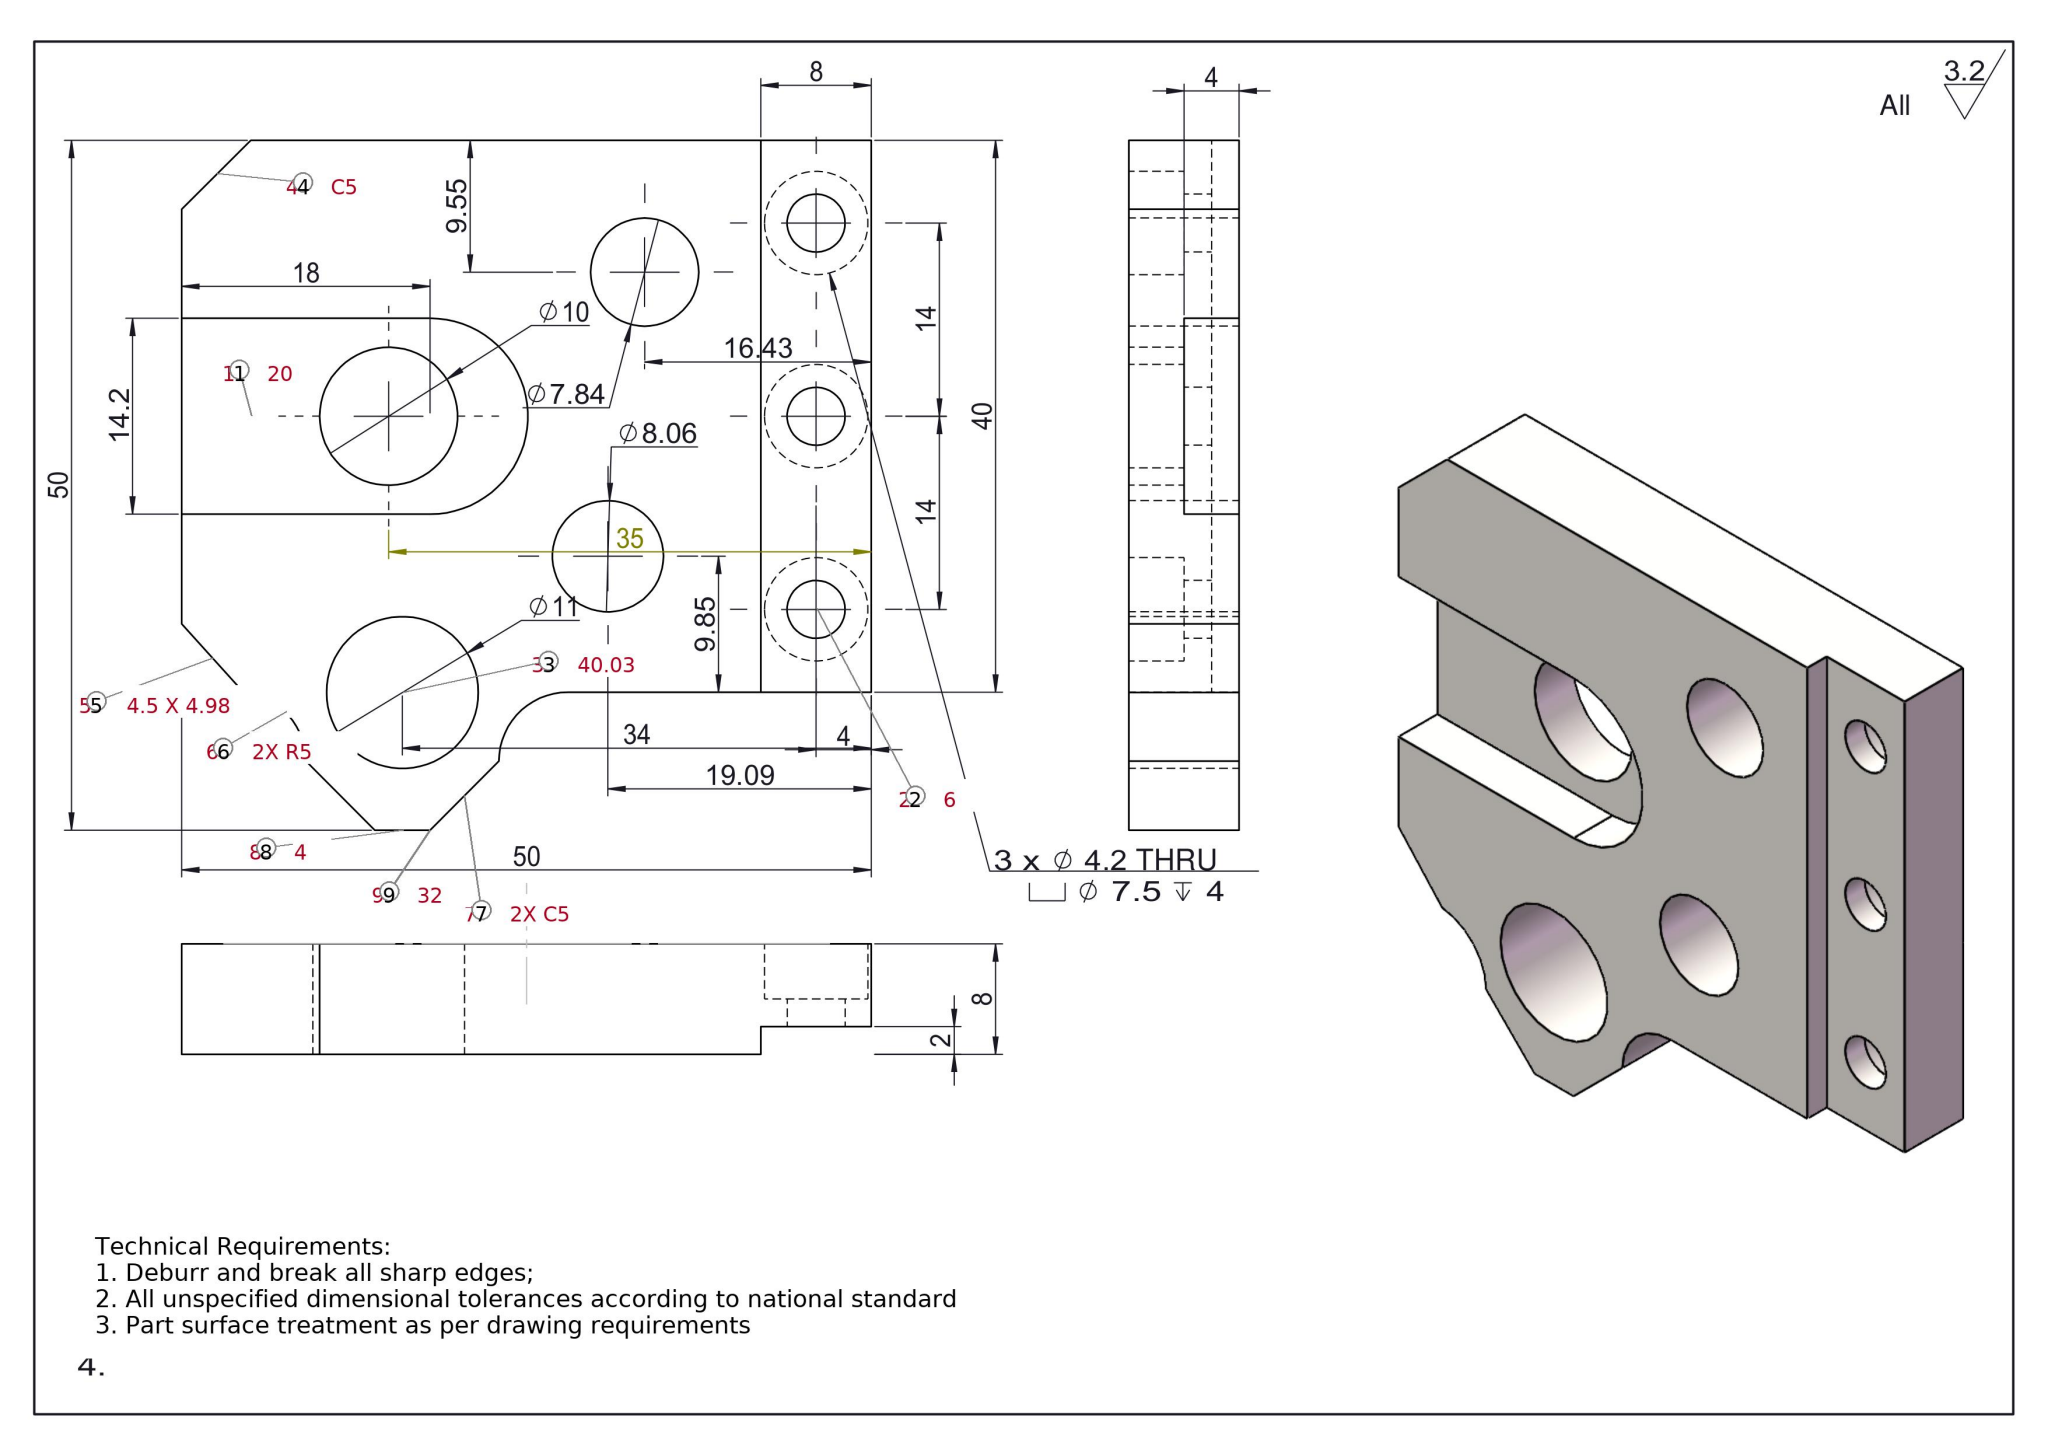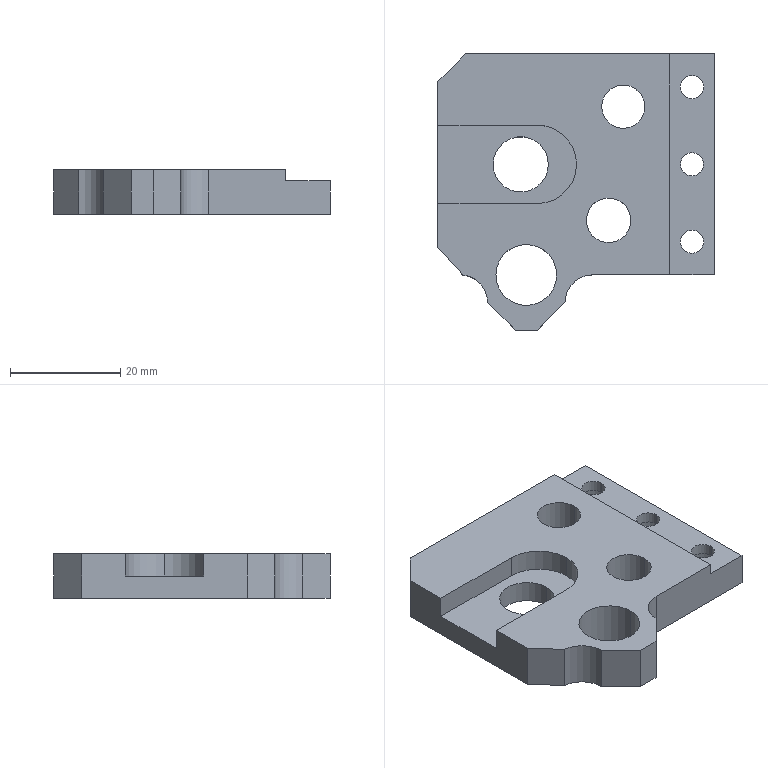Part | SolidWorks | mm | 1 solid | 43 faces | box 50 x 50 x 8 mm | volume 12357 mm3 | cylinder 24 | plane 19 | commonest cylinder face diameters 7.5 x6 4.2 x6 10 x4 8.058 x2 7.836 x2 11 x2 14.2 x2